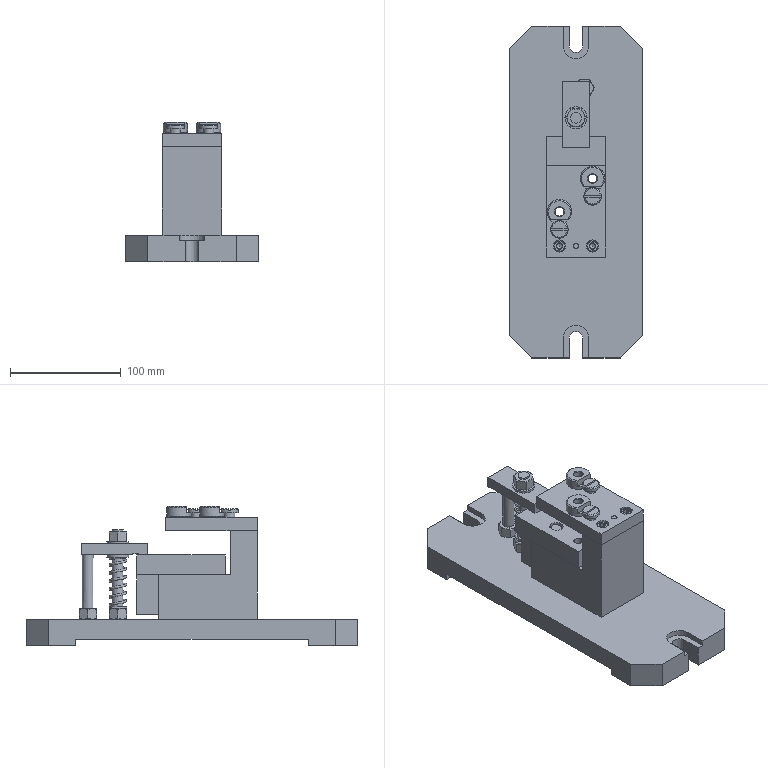Assembly | NX | mm | 21 component files | 21 solids | 358 faces | box 120 x 300 x 126 mm | volume 1092083 mm3 | plane 185 | cone 87 | cylinder 76 | spline 5 | torus 4 | sphere 1 | commonest cylinder face diameters 12 x17 10 x13 8.782 x6 11 x5 5.795 x4 8 x4 6 x4 5 x3
Bill of materials:
unnamed part 1 | 1 |  | Stepped cylindrical part shaped like a turned pin, with a wide central collar and a cylindrical section of the same diameter on each side, each section chamfered at its end
unnamed part 2 | 1 |  | Slender cylindrical pin with a domed end at one side and a flat end at the other, plus a reduced-diameter groove near the flat end
unnamed part 3 | 1 |  | Slender stepped cylindrical shaft with a reduced-diameter section at one end, ending in a thin wider lip, and a reduced-diameter groove near the other end
GB-T95-2002,M10 | 2 |  | Plain Washer, GB-T 95-2002,M10
unnamed part 4 | 2 |  | Headed pin or screw-like part with a large chamfered disc head that has a straight slot across it, a cylindrical collar under the head, a reduced neck, and a chamfered cylindrical shank
GB-T41-2000,M10x1.5 | 3 |  | Hexagonal prism with a central cylindrical through-bore and chamfered corners on both end faces; shaped like a hex nut.
unnamed part 5 | 1 |  | Flat rectangular plate with several plain round through-holes of two to three different sizes
unnamed part 6 | 2 |  | Flanged bushing-like part with a central through-bore, a chamfered round flange that has a flat cut-away step on one side, and a cylindrical shank with a chamfered end
unnamed part 7 | 1 |  | Rectangular block with a single round through-hole and shallow steps or notches on the underside
GB-T70.1-2000,M6x12 | 2 |  | Hexagon Socket Head Cap Screw, GB-T 70.1-2000,M6x12
unnamed part 8 | 1 |  | L-shaped bracket made of a rectangular top plate with four vertical through-holes and a downward leg carrying a large horizontal through-hole
GB-T119.1-2000,5x24 | 1 |  | Parallel Pin, GB-T 119.1-2000,5x24
unnamed part 9 | 1 |  | Helical coil spring of round wire with closely spaced end coils that appear flattened or ground
unnamed part 10 | 1 |  | Stepped cylindrical part with a wide central collar, a chamfered cylindrical lower end, and an upper end with parallel flats
unnamed part 11 | 1 |  | Elongated base plate with chamfered corners and an open U-slot at each end, carrying an upright stepped (L-profile) block and a pattern of round holes
Mates:
1. fix | fixture_body 1 component
2. touch align | spacer_block 1 face | fixture_body 1 face
3. center | spacer_block 1 face | spacer_block 1 face | fixture_body 1 face | fixture_body 1 face
4. touch align | spacer_block 1 face | fixture_body 1 edge
5. touch align | drill_plate 1 face | fixture_body 1 face
6. touch align | drill_plate 1 face | spacer_block 1 face
7. concentric | drill_bush 2 edge | drill_plate 1 edge
8. concentric | drill_bush_screw 2 edge | drill_plate 1 arc
9. concentric | drill_bush 1 edge | drill_plate 1 edge
10. concentric | drill_bush_screw 1 edge | drill_plate 1 arc
11. touch align | clamp_plate 1 face | spacer_block 1 face
12. touch align | fixing_screw 1 face | clamp_plate 1 face
13. center | clamp_plate 1 face | clamp_plate 1 face | fixture_body 1 face | fixture_body 1 face
14. touch align | support_screw 1 face | clamp_plate 1 face
15. touch align | support_screw 1 face | clamp_plate 1 face
16. distance | clamp_plate 1 face | fixture_body 1 face
17. concentric | GB-T95-2002_M10 2 edge | clamp_plate 1 edge
18. concentric | GB-T41-2000_M10x1_5 3 edge | GB-T95-2002_M10 2 edge
19. distance | fixing_screw 1 face | clamp_plate 1 face
20. concentric | GB-T41-2000_M10x1_5 1 edge | fixture_body 1 arc
21. concentric | GB-T41-2000_M10x1_5 2 edge | fixture_body 1 arc
22. touch align | GB-T95-2002_M10 1 face | fixing_screw 1 face
23. touch align | GB-T95-2002_M10 1 face | clamp_plate 1 face
24. concentric | spring 1 edge | GB-T41-2000_M10x1_5 1 edge
25. concentric | A_locating_pin 1 edge | fixture_body 1 edge
26. concentric | B_locating_pin 1 edge | fixture_body 1 edge